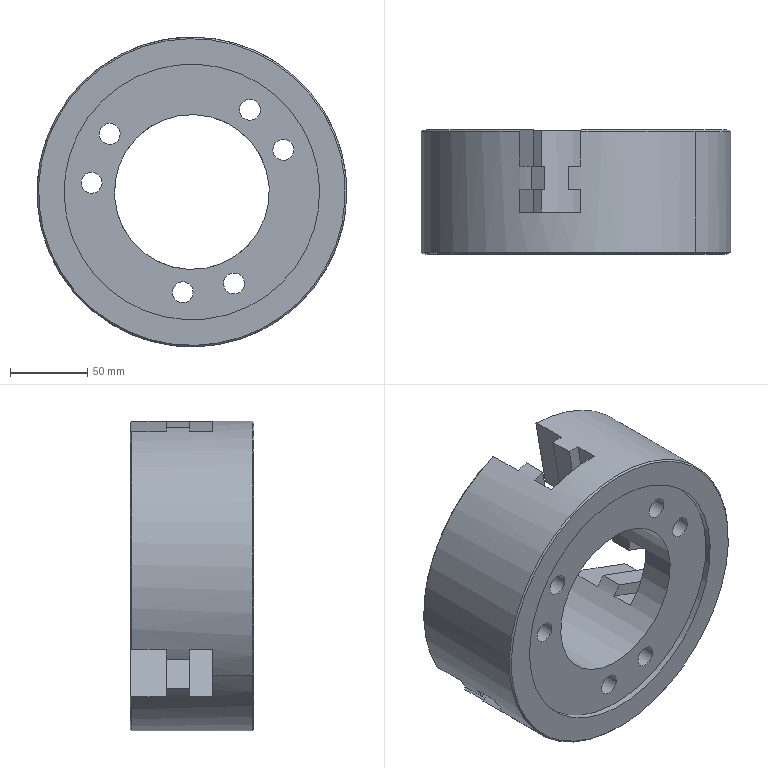Component | SolidWorks | K51-2_K51-1-1 | 1 solid | 79 faces | volume 1462041 mm3 | plane 44 | cylinder 30 | cone 5 | commonest cylinder face diameters 20 x12 13.5 x12 165 x2 200 x2 100 x2